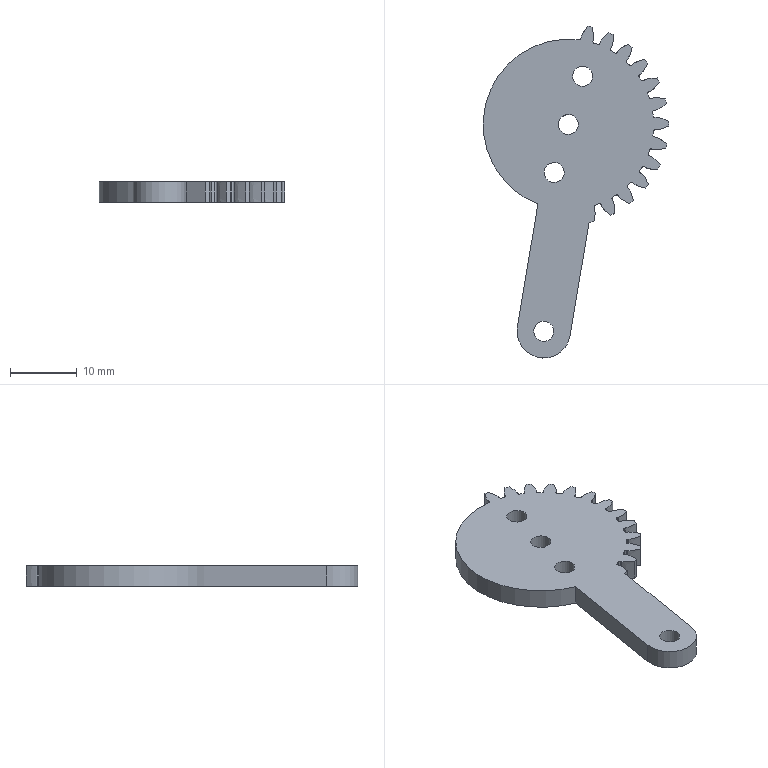Component | NX | GEAR-LINK-2_YEN | 1 solid | 111 faces | volume 2100 mm3 | cylinder 56 | plane 29 | other 26 | commonest cylinder face diameters 0.5 x25 30 x13 25.5 x13 3 x4 8 x1